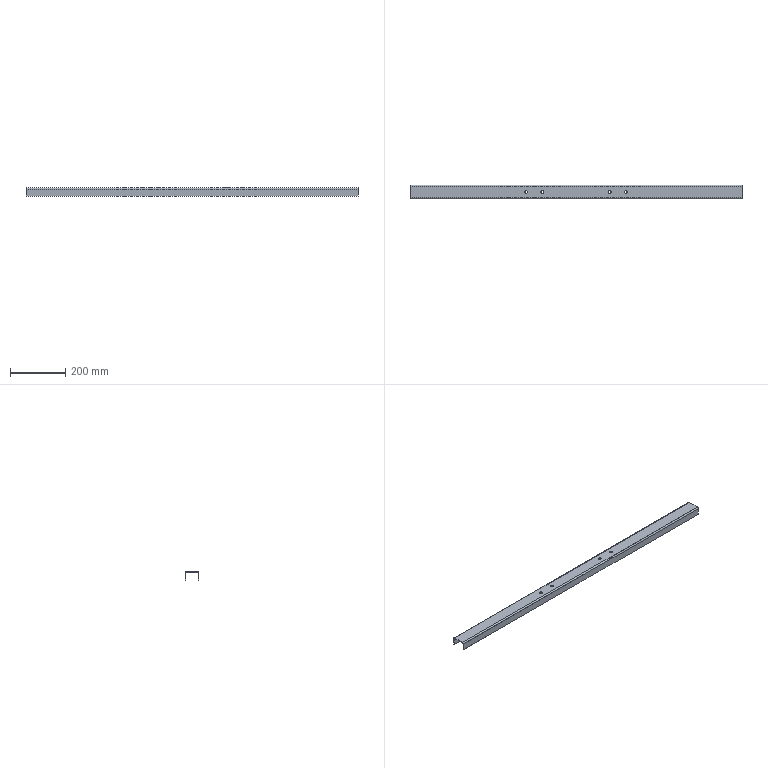Component | SolidWorks | 50x30x2ColdBentEqualAngleSteel1200mm-1 | 1 solid | 22 faces | box 1200 x 50 x 30 mm | volume 245531 mm3 | cylinder 12 | plane 10 | commonest cylinder face diameters 10 x10 6 x2
build123d program:
from build123d import *

# Parameters (mm, degrees)
BOSS_EXTRUDE1_DEPTH = 1200
SKETCH2_R           = 5
CUT_EXTRUDE1_DEPTH  = 10


with BuildPart() as part:
    # Sketch1 → Boss-Extrude1 (new body)
    with BuildSketch(Plane(origin=(0, 0, 0), x_dir=(0, 0, -1), z_dir=(1, 0, 0))):
        with BuildLine():
            Line((0, 5), (0, 45))
            ThreePointArc((0, 45), (1.464, 48.536), (5, 50))
            Line((5, 50), (30, 50))
            Line((30, 50), (30, 48))
            Line((30, 48), (5, 48))
            ThreePointArc((5, 48), (2.879, 47.121), (2, 45))
            Line((2, 45), (2, 5))
            ThreePointArc((2, 5), (2.879, 2.879), (5, 2))
            Line((5, 2), (30, 2))
            Line((30, 2), (30, 0))
            Line((30, 0), (5, 0))
            ThreePointArc((5, 0), (1.464, 1.464), (0, 5))
        make_face()
    extrude(amount=BOSS_EXTRUDE1_DEPTH)

    # Sketch2 → Cut-Extrude1 (cut)
    with BuildSketch(Plane.XY):
        with Locations((420, 25)):
            Circle(SKETCH2_R)
        with Locations((478, 25)):
            Circle(SKETCH2_R)
    cut_extrude1 = extrude(amount=-CUT_EXTRUDE1_DEPTH, mode=Mode.SUBTRACT)

    # Mirror2: Cut-Extrude1 across plane
    add(cut_extrude1.mirror(Plane.ZY.offset(-600)), mode=Mode.SUBTRACT)


solid = part.part

# Placed as in the assembly
solid = solid.moved(Location((-574.371, -297.9, 415), (0, 0, 0)))
STEP:
#1=COLOUR_RGB('',0.7922,0.8196,0.9333);
#2=FILL_AREA_STYLE_COLOUR('',#1);
#3=FILL_AREA_STYLE('',(#2));
#4=SURFACE_STYLE_FILL_AREA(#3);
#5=SURFACE_SIDE_STYLE('',(#4));
#6=SURFACE_STYLE_USAGE(.BOTH.,#5);
#7=PRESENTATION_STYLE_ASSIGNMENT((#6));
#8=CARTESIAN_POINT('',(8.292,-10.744,16.26));
#9=VERTEX_POINT('',#8);
#10=CARTESIAN_POINT('',(7.899,-10.744,16.26));
#11=VERTEX_POINT('',#10);
#12=CARTESIAN_POINT('',(8.096,-10.744,16.26));
#13=DIRECTION('',(0.,0.,-1.));
#14=DIRECTION('',(1.,0.,0.));
#15=AXIS2_PLACEMENT_3D('',#12,#13,#14);
#16=CIRCLE('',#15,0.1969);
#17=EDGE_CURVE('',#9,#11,#16,.T.);
#18=ORIENTED_EDGE('',*,*,#17,.T.);
#19=CARTESIAN_POINT('',(7.899,-10.744,16.339));
#20=VERTEX_POINT('',#19);
#21=CARTESIAN_POINT('',(7.899,-10.744,15.945));
#22=DIRECTION('',(0.,0.,1.));
#23=VECTOR('',#22,39.37);
#24=LINE('',#21,#23);
#25=EDGE_CURVE('',#11,#20,#24,.T.);
#26=ORIENTED_EDGE('',*,*,#25,.T.);
#27=CARTESIAN_POINT('',(8.292,-10.744,16.339));
#28=VERTEX_POINT('',#27);
#29=CARTESIAN_POINT('',(8.096,-10.744,16.339));
#30=DIRECTION('',(0.,0.,-1.));
#31=DIRECTION('',(-1.,0.,0.));
#32=AXIS2_PLACEMENT_3D('',#29,#30,#31);
#33=CIRCLE('',#32,0.1969);
#34=EDGE_CURVE('',#28,#20,#33,.T.);
#35=ORIENTED_EDGE('',*,*,#34,.F.);
#36=CARTESIAN_POINT('',(8.292,-10.744,15.945));
#37=DIRECTION('',(0.,0.,1.));
#38=VECTOR('',#37,39.37);
#39=LINE('',#36,#38);
#40=EDGE_CURVE('',#9,#28,#39,.T.);
#41=ORIENTED_EDGE('',*,*,#40,.F.);
#42=EDGE_LOOP('',(#18,#26,#35,#41));
#43=FACE_OUTER_BOUND('',#42,.T.);
#44=CARTESIAN_POINT('',(8.096,-10.744,15.945));
#45=DIRECTION('',(0.,0.,1.));
#46=DIRECTION('',(1.,0.,0.));
#47=AXIS2_PLACEMENT_3D('',#44,#45,#46);
#48=CYLINDRICAL_SURFACE('',#47,0.1969);
#49=ADVANCED_FACE('',(#43),#48,.F.);
#50=CARTESIAN_POINT('',(6.009,-10.744,16.26));
#51=VERTEX_POINT('',#50);
#52=CARTESIAN_POINT('',(5.615,-10.744,16.26));
#53=VERTEX_POINT('',#52);
#54=CARTESIAN_POINT('',(5.812,-10.744,16.26));
#55=DIRECTION('',(0.,0.,-1.));
#56=DIRECTION('',(1.,0.,0.));
#57=AXIS2_PLACEMENT_3D('',#54,#55,#56);
#58=CIRCLE('',#57,0.1969);
#59=EDGE_CURVE('',#51,#53,#58,.T.);
#60=ORIENTED_EDGE('',*,*,#59,.T.);
#61=CARTESIAN_POINT('',(5.615,-10.744,16.339));
#62=VERTEX_POINT('',#61);
#63=CARTESIAN_POINT('',(5.615,-10.744,15.945));
#64=DIRECTION('',(0.,0.,1.));
#65=VECTOR('',#64,39.37);
#66=LINE('',#63,#65);
#67=EDGE_CURVE('',#53,#62,#66,.T.);
#68=ORIENTED_EDGE('',*,*,#67,.T.);
#69=CARTESIAN_POINT('',(6.009,-10.744,16.339));
#70=VERTEX_POINT('',#69);
#71=CARTESIAN_POINT('',(5.812,-10.744,16.339));
#72=DIRECTION('',(0.,0.,-1.));
#73=DIRECTION('',(-1.,0.,0.));
#74=AXIS2_PLACEMENT_3D('',#71,#72,#73);
#75=CIRCLE('',#74,0.1969);
#76=EDGE_CURVE('',#70,#62,#75,.T.);
#77=ORIENTED_EDGE('',*,*,#76,.F.);
#78=CARTESIAN_POINT('',(6.009,-10.744,15.945));
#79=DIRECTION('',(0.,0.,1.));
#80=VECTOR('',#79,39.37);
#81=LINE('',#78,#80);
#82=EDGE_CURVE('',#51,#70,#81,.T.);
#83=ORIENTED_EDGE('',*,*,#82,.F.);
#84=EDGE_LOOP('',(#60,#68,#77,#83));
#85=FACE_OUTER_BOUND('',#84,.T.);
#86=CARTESIAN_POINT('',(5.812,-10.744,15.945));
#87=DIRECTION('',(0.,0.,1.));
#88=DIRECTION('',(1.,0.,0.));
#89=AXIS2_PLACEMENT_3D('',#86,#87,#88);
#90=CYLINDRICAL_SURFACE('',#89,0.1969);
#91=ADVANCED_FACE('',(#85),#90,.F.);
#92=CARTESIAN_POINT('',(-6.274,-10.744,16.26));
#93=VERTEX_POINT('',#92);
#94=CARTESIAN_POINT('',(-5.881,-10.744,16.26));
#95=VERTEX_POINT('',#94);
#96=CARTESIAN_POINT('',(-6.078,-10.744,16.26));
#97=DIRECTION('',(0.,0.,1.));
#98=DIRECTION('',(1.,0.,0.));
#99=AXIS2_PLACEMENT_3D('',#96,#97,#98);
#100=CIRCLE('',#99,0.1969);
#101=EDGE_CURVE('',#93,#95,#100,.T.);
#102=ORIENTED_EDGE('',*,*,#101,.F.);
#103=CARTESIAN_POINT('',(-6.274,-10.744,16.339));
#104=VERTEX_POINT('',#103);
#105=CARTESIAN_POINT('',(-6.274,-10.744,15.945));
#106=DIRECTION('',(0.,0.,1.));
#107=VECTOR('',#106,39.37);
#108=LINE('',#105,#107);
#109=EDGE_CURVE('',#93,#104,#108,.T.);
#110=ORIENTED_EDGE('',*,*,#109,.T.);
#111=CARTESIAN_POINT('',(-5.881,-10.744,16.339));
#112=VERTEX_POINT('',#111);
#113=CARTESIAN_POINT('',(-6.078,-10.744,16.339));
#114=DIRECTION('',(0.,0.,1.));
#115=DIRECTION('',(1.,0.,0.));
#116=AXIS2_PLACEMENT_3D('',#113,#114,#115);
#117=CIRCLE('',#116,0.1969);
#118=EDGE_CURVE('',#104,#112,#117,.T.);
#119=ORIENTED_EDGE('',*,*,#118,.T.);
#120=CARTESIAN_POINT('',(-5.881,-10.744,15.945));
#121=DIRECTION('',(0.,0.,1.));
#122=VECTOR('',#121,39.37);
#123=LINE('',#120,#122);
#124=EDGE_CURVE('',#95,#112,#123,.T.);
#125=ORIENTED_EDGE('',*,*,#124,.F.);
#126=EDGE_LOOP('',(#102,#110,#119,#125));
#127=FACE_OUTER_BOUND('',#126,.T.);
#128=CARTESIAN_POINT('',(-6.078,-10.744,15.945));
#129=DIRECTION('',(0.,0.,1.));
#130=DIRECTION('',(1.,0.,0.));
#131=AXIS2_PLACEMENT_3D('',#128,#129,#130);
#132=CYLINDRICAL_SURFACE('',#131,0.1969);
#133=ADVANCED_FACE('',(#127),#132,.F.);
#134=CARTESIAN_POINT('',(-3.991,-10.744,16.26));
#135=VERTEX_POINT('',#134);
#136=CARTESIAN_POINT('',(-3.597,-10.744,16.26));
#137=VERTEX_POINT('',#136);
#138=CARTESIAN_POINT('',(-3.794,-10.744,16.26));
#139=DIRECTION('',(0.,0.,1.));
#140=DIRECTION('',(1.,0.,0.));
#141=AXIS2_PLACEMENT_3D('',#138,#139,#140);
#142=CIRCLE('',#141,0.1969);
#143=EDGE_CURVE('',#135,#137,#142,.T.);
#144=ORIENTED_EDGE('',*,*,#143,.F.);
#145=CARTESIAN_POINT('',(-3.991,-10.744,16.339));
#146=VERTEX_POINT('',#145);
#147=CARTESIAN_POINT('',(-3.991,-10.744,15.945));
#148=DIRECTION('',(0.,0.,1.));
#149=VECTOR('',#148,39.37);
#150=LINE('',#147,#149);
#151=EDGE_CURVE('',#135,#146,#150,.T.);
#152=ORIENTED_EDGE('',*,*,#151,.T.);
#153=CARTESIAN_POINT('',(-3.597,-10.744,16.339));
#154=VERTEX_POINT('',#153);
#155=CARTESIAN_POINT('',(-3.794,-10.744,16.339));
#156=DIRECTION('',(0.,0.,1.));
#157=DIRECTION('',(1.,0.,0.));
#158=AXIS2_PLACEMENT_3D('',#155,#156,#157);
#159=CIRCLE('',#158,0.1969);
#160=EDGE_CURVE('',#146,#154,#159,.T.);
#161=ORIENTED_EDGE('',*,*,#160,.T.);
#162=CARTESIAN_POINT('',(-3.597,-10.744,15.945));
#163=DIRECTION('',(0.,0.,1.));
#164=VECTOR('',#163,39.37);
#165=LINE('',#162,#164);
#166=EDGE_CURVE('',#137,#154,#165,.T.);
#167=ORIENTED_EDGE('',*,*,#166,.F.);
#168=EDGE_LOOP('',(#144,#152,#161,#167));
#169=FACE_OUTER_BOUND('',#168,.T.);
#170=CARTESIAN_POINT('',(-3.794,-10.744,15.945));
#171=DIRECTION('',(0.,0.,1.));
#172=DIRECTION('',(1.,0.,0.));
#173=AXIS2_PLACEMENT_3D('',#170,#171,#172);
#174=CYLINDRICAL_SURFACE('',#173,0.1969);
#175=ADVANCED_FACE('',(#169),#174,.F.);
#176=CARTESIAN_POINT('',(-22.613,-9.76,16.142));
#177=VERTEX_POINT('',#176);
#178=CARTESIAN_POINT('',(-22.613,-9.957,16.339));
#179=VERTEX_POINT('',#178);
#180=CARTESIAN_POINT('',(-22.613,-9.957,16.142));
#181=DIRECTION('',(1.,0.,0.));
#182=DIRECTION('',(0.,0.,1.));
#183=AXIS2_PLACEMENT_3D('',#180,#181,#182);
#184=CIRCLE('',#183,0.1969);
#185=EDGE_CURVE('',#177,#179,#184,.T.);
#186=ORIENTED_EDGE('',*,*,#185,.T.);
#187=CARTESIAN_POINT('',(24.631,-9.957,16.339));
#188=VERTEX_POINT('',#187);
#189=CARTESIAN_POINT('',(24.631,-9.957,16.339));
#190=DIRECTION('',(-1.,0.,0.));
#191=VECTOR('',#190,39.37);
#192=LINE('',#189,#191);
#193=EDGE_CURVE('',#188,#179,#192,.T.);
#194=ORIENTED_EDGE('',*,*,#193,.F.);
#195=CARTESIAN_POINT('',(24.631,-9.76,16.142));
#196=VERTEX_POINT('',#195);
#197=CARTESIAN_POINT('',(24.631,-9.957,16.142));
#198=DIRECTION('',(1.,0.,0.));
#199=DIRECTION('',(0.,0.,1.));
#200=AXIS2_PLACEMENT_3D('',#197,#198,#199);
#201=CIRCLE('',#200,0.1969);
#202=EDGE_CURVE('',#196,#188,#201,.T.);
#203=ORIENTED_EDGE('',*,*,#202,.F.);
#204=CARTESIAN_POINT('',(24.631,-9.76,16.142));
#205=DIRECTION('',(-1.,0.,0.));
#206=VECTOR('',#205,39.37);
#207=LINE('',#204,#206);
#208=EDGE_CURVE('',#196,#177,#207,.T.);
#209=ORIENTED_EDGE('',*,*,#208,.T.);
#210=EDGE_LOOP('',(#186,#194,#203,#209));
#211=FACE_OUTER_BOUND('',#210,.T.);
#212=CARTESIAN_POINT('',(24.631,-9.957,16.142));
#213=DIRECTION('',(-1.,0.,0.));
#214=DIRECTION('',(0.,0.,1.));
#215=AXIS2_PLACEMENT_3D('',#212,#213,#214);
#216=CYLINDRICAL_SURFACE('',#215,0.1969);
#217=ADVANCED_FACE('',(#211),#216,.T.);
#218=ORIENTED_EDGE('',*,*,#34,.T.);
#219=CARTESIAN_POINT('',(8.096,-10.744,16.339));
#220=DIRECTION('',(0.,0.,-1.));
#221=DIRECTION('',(-1.,0.,0.));
#222=AXIS2_PLACEMENT_3D('',#219,#220,#221);
#223=CIRCLE('',#222,0.1969);
#224=EDGE_CURVE('',#20,#28,#223,.T.);
#225=ORIENTED_EDGE('',*,*,#224,.T.);
#226=EDGE_LOOP('',(#218,#225));
#227=FACE_BOUND('',#226,.T.);
#228=ORIENTED_EDGE('',*,*,#76,.T.);
#229=CARTESIAN_POINT('',(5.812,-10.744,16.339));
#230=DIRECTION('',(0.,0.,-1.));
#231=DIRECTION('',(-1.,0.,0.));
#232=AXIS2_PLACEMENT_3D('',#229,#230,#231);
#233=CIRCLE('',#232,0.1969);
#234=EDGE_CURVE('',#62,#70,#233,.T.);
#235=ORIENTED_EDGE('',*,*,#234,.T.);
#236=EDGE_LOOP('',(#228,#235));
#237=FACE_BOUND('',#236,.T.);
#238=CARTESIAN_POINT('',(-6.078,-10.744,16.339));
#239=DIRECTION('',(0.,0.,1.));
#240=DIRECTION('',(1.,0.,0.));
#241=AXIS2_PLACEMENT_3D('',#238,#239,#240);
#242=CIRCLE('',#241,0.1969);
#243=EDGE_CURVE('',#112,#104,#242,.T.);
#244=ORIENTED_EDGE('',*,*,#243,.F.);
#245=ORIENTED_EDGE('',*,*,#118,.F.);
#246=EDGE_LOOP('',(#244,#245));
#247=FACE_BOUND('',#246,.T.);
#248=CARTESIAN_POINT('',(-3.794,-10.744,16.339));
#249=DIRECTION('',(0.,0.,1.));
#250=DIRECTION('',(1.,0.,0.));
#251=AXIS2_PLACEMENT_3D('',#248,#249,#250);
#252=CIRCLE('',#251,0.1969);
#253=EDGE_CURVE('',#154,#146,#252,.T.);
#254=ORIENTED_EDGE('',*,*,#253,.F.);
#255=ORIENTED_EDGE('',*,*,#160,.F.);
#256=EDGE_LOOP('',(#254,#255));
#257=FACE_BOUND('',#256,.T.);
#258=CARTESIAN_POINT('',(-22.613,-11.532,16.339));
#259=VERTEX_POINT('',#258);
#260=CARTESIAN_POINT('',(-22.613,-11.532,16.339));
#261=DIRECTION('',(0.,-1.,0.));
#262=VECTOR('',#261,39.37);
#263=LINE('',#260,#262);
#264=EDGE_CURVE('',#179,#259,#263,.T.);
#265=ORIENTED_EDGE('',*,*,#264,.T.);
#266=CARTESIAN_POINT('',(24.631,-11.532,16.339));
#267=VERTEX_POINT('',#266);
#268=CARTESIAN_POINT('',(24.631,-11.532,16.339));
#269=DIRECTION('',(-1.,0.,0.));
#270=VECTOR('',#269,39.37);
#271=LINE('',#268,#270);
#272=EDGE_CURVE('',#267,#259,#271,.T.);
#273=ORIENTED_EDGE('',*,*,#272,.F.);
#274=CARTESIAN_POINT('',(24.631,-11.532,16.339));
#275=DIRECTION('',(0.,-1.,0.));
#276=VECTOR('',#275,39.37);
#277=LINE('',#274,#276);
#278=EDGE_CURVE('',#188,#267,#277,.T.);
#279=ORIENTED_EDGE('',*,*,#278,.F.);
#280=ORIENTED_EDGE('',*,*,#193,.T.);
#281=EDGE_LOOP('',(#265,#273,#279,#280));
#282=FACE_OUTER_BOUND('',#281,.T.);
#283=CARTESIAN_POINT('',(24.631,-11.532,16.339));
#284=DIRECTION('',(0.,0.,-1.));
#285=DIRECTION('',(-1.,0.,0.));
#286=AXIS2_PLACEMENT_3D('',#283,#284,#285);
#287=PLANE('',#286);
#288=ADVANCED_FACE('',(#227,#237,#247,#257,#282),#287,.F.);
#289=CARTESIAN_POINT('',(-22.613,-11.728,16.142));
#290=VERTEX_POINT('',#289);
#291=CARTESIAN_POINT('',(-22.613,-11.532,16.142));
#292=DIRECTION('',(1.,0.,0.));
#293=DIRECTION('',(0.,0.,-1.));
#294=AXIS2_PLACEMENT_3D('',#291,#292,#293);
#295=CIRCLE('',#294,0.1969);
#296=EDGE_CURVE('',#259,#290,#295,.T.);
#297=ORIENTED_EDGE('',*,*,#296,.T.);
#298=CARTESIAN_POINT('',(24.631,-11.728,16.142));
#299=VERTEX_POINT('',#298);
#300=CARTESIAN_POINT('',(24.631,-11.728,16.142));
#301=DIRECTION('',(-1.,0.,0.));
#302=VECTOR('',#301,39.37);
#303=LINE('',#300,#302);
#304=EDGE_CURVE('',#299,#290,#303,.T.);
#305=ORIENTED_EDGE('',*,*,#304,.F.);
#306=CARTESIAN_POINT('',(24.631,-11.532,16.142));
#307=DIRECTION('',(1.,0.,0.));
#308=DIRECTION('',(0.,0.,-1.));
#309=AXIS2_PLACEMENT_3D('',#306,#307,#308);
#310=CIRCLE('',#309,0.1969);
#311=EDGE_CURVE('',#267,#299,#310,.T.);
#312=ORIENTED_EDGE('',*,*,#311,.F.);
#313=ORIENTED_EDGE('',*,*,#272,.T.);
#314=EDGE_LOOP('',(#297,#305,#312,#313));
#315=FACE_OUTER_BOUND('',#314,.T.);
#316=CARTESIAN_POINT('',(24.631,-11.532,16.142));
#317=DIRECTION('',(-1.,0.,0.));
#318=DIRECTION('',(0.,0.,1.));
#319=AXIS2_PLACEMENT_3D('',#316,#317,#318);
#320=CYLINDRICAL_SURFACE('',#319,0.1969);
#321=ADVANCED_FACE('',(#315),#320,.T.);
#322=CARTESIAN_POINT('',(-22.613,-11.728,15.157));
#323=VERTEX_POINT('',#322);
#324=CARTESIAN_POINT('',(-22.613,-11.728,16.142));
#325=DIRECTION('',(0.,0.,-1.));
#326=VECTOR('',#325,39.37);
#327=LINE('',#324,#326);
#328=EDGE_CURVE('',#290,#323,#327,.T.);
#329=ORIENTED_EDGE('',*,*,#328,.T.);
#330=CARTESIAN_POINT('',(24.631,-11.728,15.157));
#331=VERTEX_POINT('',#330);
#332=CARTESIAN_POINT('',(24.631,-11.728,15.157));
#333=DIRECTION('',(-1.,0.,0.));
#334=VECTOR('',#333,39.37);
#335=LINE('',#332,#334);
#336=EDGE_CURVE('',#331,#323,#335,.T.);
#337=ORIENTED_EDGE('',*,*,#336,.F.);
#338=CARTESIAN_POINT('',(24.631,-11.728,16.142));
#339=DIRECTION('',(0.,0.,-1.));
#340=VECTOR('',#339,39.37);
#341=LINE('',#338,#340);
#342=EDGE_CURVE('',#299,#331,#341,.T.);
#343=ORIENTED_EDGE('',*,*,#342,.F.);
#344=ORIENTED_EDGE('',*,*,#304,.T.);
#345=EDGE_LOOP('',(#329,#337,#343,#344));
#346=FACE_OUTER_BOUND('',#345,.T.);
#347=CARTESIAN_POINT('',(24.631,-11.728,16.142));
#348=DIRECTION('',(0.,1.,0.));
#349=DIRECTION('',(0.,0.,1.));
#350=AXIS2_PLACEMENT_3D('',#347,#348,#349);
#351=PLANE('',#350);
#352=ADVANCED_FACE('',(#346),#351,.F.);
#353=CARTESIAN_POINT('',(-22.613,-11.65,15.157));
#354=VERTEX_POINT('',#353);
#355=CARTESIAN_POINT('',(-22.613,-11.65,15.157));
#356=DIRECTION('',(0.,1.,0.));
#357=VECTOR('',#356,39.37);
#358=LINE('',#355,#357);
#359=EDGE_CURVE('',#323,#354,#358,.T.);
#360=ORIENTED_EDGE('',*,*,#359,.T.);
#361=CARTESIAN_POINT('',(24.631,-11.65,15.157));
#362=VERTEX_POINT('',#361);
#363=CARTESIAN_POINT('',(24.631,-11.65,15.157));
#364=DIRECTION('',(-1.,0.,0.));
#365=VECTOR('',#364,39.37);
#366=LINE('',#363,#365);
#367=EDGE_CURVE('',#362,#354,#366,.T.);
#368=ORIENTED_EDGE('',*,*,#367,.F.);
#369=CARTESIAN_POINT('',(24.631,-11.65,15.157));
#370=DIRECTION('',(0.,1.,0.));
#371=VECTOR('',#370,39.37);
#372=LINE('',#369,#371);
#373=EDGE_CURVE('',#331,#362,#372,.T.);
#374=ORIENTED_EDGE('',*,*,#373,.F.);
#375=ORIENTED_EDGE('',*,*,#336,.T.);
#376=EDGE_LOOP('',(#360,#368,#374,#375));
#377=FACE_OUTER_BOUND('',#376,.T.);
#378=CARTESIAN_POINT('',(24.631,-11.65,15.157));
#379=DIRECTION('',(0.,0.,1.));
#380=DIRECTION('',(1.,0.,0.));
#381=AXIS2_PLACEMENT_3D('',#378,#379,#380);
#382=PLANE('',#381);
#383=ADVANCED_FACE('',(#377),#382,.F.);
#384=CARTESIAN_POINT('',(-22.613,-11.65,16.142));
#385=VERTEX_POINT('',#384);
#386=CARTESIAN_POINT('',(-22.613,-11.65,16.142));
#387=DIRECTION('',(0.,0.,1.));
#388=VECTOR('',#387,39.37);
#389=LINE('',#386,#388);
#390=EDGE_CURVE('',#354,#385,#389,.T.);
#391=ORIENTED_EDGE('',*,*,#390,.T.);
#392=CARTESIAN_POINT('',(24.631,-11.65,16.142));
#393=VERTEX_POINT('',#392);
#394=CARTESIAN_POINT('',(24.631,-11.65,16.142));
#395=DIRECTION('',(-1.,0.,0.));
#396=VECTOR('',#395,39.37);
#397=LINE('',#394,#396);
#398=EDGE_CURVE('',#393,#385,#397,.T.);
#399=ORIENTED_EDGE('',*,*,#398,.F.);
#400=CARTESIAN_POINT('',(24.631,-11.65,16.142));
#401=DIRECTION('',(0.,0.,1.));
#402=VECTOR('',#401,39.37);
#403=LINE('',#400,#402);
#404=EDGE_CURVE('',#362,#393,#403,.T.);
#405=ORIENTED_EDGE('',*,*,#404,.F.);
#406=ORIENTED_EDGE('',*,*,#367,.T.);
#407=EDGE_LOOP('',(#391,#399,#405,#406));
#408=FACE_OUTER_BOUND('',#407,.T.);
#409=CARTESIAN_POINT('',(24.631,-11.65,16.142));
#410=DIRECTION('',(0.,-1.,0.));
#411=DIRECTION('',(0.,0.,-1.));
#412=AXIS2_PLACEMENT_3D('',#409,#410,#411);
#413=PLANE('',#412);
#414=ADVANCED_FACE('',(#408),#413,.F.);
#415=CARTESIAN_POINT('',(-22.613,-11.532,16.26));
#416=VERTEX_POINT('',#415);
#417=CARTESIAN_POINT('',(-22.613,-11.532,16.142));
#418=DIRECTION('',(-1.,0.,0.));
#419=DIRECTION('',(0.,0.,-1.));
#420=AXIS2_PLACEMENT_3D('',#417,#418,#419);
#421=CIRCLE('',#420,0.1181);
#422=EDGE_CURVE('',#385,#416,#421,.T.);
#423=ORIENTED_EDGE('',*,*,#422,.T.);
#424=CARTESIAN_POINT('',(24.631,-11.532,16.26));
#425=VERTEX_POINT('',#424);
#426=CARTESIAN_POINT('',(24.631,-11.532,16.26));
#427=DIRECTION('',(-1.,0.,0.));
#428=VECTOR('',#427,39.37);
#429=LINE('',#426,#428);
#430=EDGE_CURVE('',#425,#416,#429,.T.);
#431=ORIENTED_EDGE('',*,*,#430,.F.);
#432=CARTESIAN_POINT('',(24.631,-11.532,16.142));
#433=DIRECTION('',(-1.,0.,0.));
#434=DIRECTION('',(0.,0.,-1.));
#435=AXIS2_PLACEMENT_3D('',#432,#433,#434);
#436=CIRCLE('',#435,0.1181);
#437=EDGE_CURVE('',#393,#425,#436,.T.);
#438=ORIENTED_EDGE('',*,*,#437,.F.);
#439=ORIENTED_EDGE('',*,*,#398,.T.);
#440=EDGE_LOOP('',(#423,#431,#438,#439));
#441=FACE_OUTER_BOUND('',#440,.T.);
#442=CARTESIAN_POINT('',(24.631,-11.532,16.142));
#443=DIRECTION('',(-1.,0.,0.));
#444=DIRECTION('',(0.,0.,1.));
#445=AXIS2_PLACEMENT_3D('',#442,#443,#444);
#446=CYLINDRICAL_SURFACE('',#445,0.1181);
#447=ADVANCED_FACE('',(#441),#446,.F.);
#448=ORIENTED_EDGE('',*,*,#17,.F.);
#449=CARTESIAN_POINT('',(8.096,-10.744,16.26));
#450=DIRECTION('',(0.,0.,-1.));
#451=DIRECTION('',(1.,0.,0.));
#452=AXIS2_PLACEMENT_3D('',#449,#450,#451);
#453=CIRCLE('',#452,0.1969);
#454=EDGE_CURVE('',#11,#9,#453,.T.);
#455=ORIENTED_EDGE('',*,*,#454,.F.);
#456=EDGE_LOOP('',(#448,#455));
#457=FACE_BOUND('',#456,.T.);
#458=ORIENTED_EDGE('',*,*,#59,.F.);
#459=CARTESIAN_POINT('',(5.812,-10.744,16.26));
#460=DIRECTION('',(0.,0.,-1.));
#461=DIRECTION('',(1.,0.,0.));
#462=AXIS2_PLACEMENT_3D('',#459,#460,#461);
#463=CIRCLE('',#462,0.1969);
#464=EDGE_CURVE('',#53,#51,#463,.T.);
#465=ORIENTED_EDGE('',*,*,#464,.F.);
#466=EDGE_LOOP('',(#458,#465));
#467=FACE_BOUND('',#466,.T.);
#468=CARTESIAN_POINT('',(-6.078,-10.744,16.26));
#469=DIRECTION('',(0.,0.,1.));
#470=DIRECTION('',(1.,0.,0.));
#471=AXIS2_PLACEMENT_3D('',#468,#469,#470);
#472=CIRCLE('',#471,0.1969);
#473=EDGE_CURVE('',#95,#93,#472,.T.);
#474=ORIENTED_EDGE('',*,*,#473,.T.);
#475=ORIENTED_EDGE('',*,*,#101,.T.);
#476=EDGE_LOOP('',(#474,#475));
#477=FACE_BOUND('',#476,.T.);
#478=CARTESIAN_POINT('',(-3.794,-10.744,16.26));
#479=DIRECTION('',(0.,0.,1.));
#480=DIRECTION('',(1.,0.,0.));
#481=AXIS2_PLACEMENT_3D('',#478,#479,#480);
#482=CIRCLE('',#481,0.1969);
#483=EDGE_CURVE('',#137,#135,#482,.T.);
#484=ORIENTED_EDGE('',*,*,#483,.T.);
#485=ORIENTED_EDGE('',*,*,#143,.T.);
#486=EDGE_LOOP('',(#484,#485));
#487=FACE_BOUND('',#486,.T.);
#488=CARTESIAN_POINT('',(-22.613,-9.957,16.26));
#489=VERTEX_POINT('',#488);
#490=CARTESIAN_POINT('',(-22.613,-11.532,16.26));
#491=DIRECTION('',(0.,1.,0.));
#492=VECTOR('',#491,39.37);
#493=LINE('',#490,#492);
#494=EDGE_CURVE('',#416,#489,#493,.T.);
#495=ORIENTED_EDGE('',*,*,#494,.T.);
#496=CARTESIAN_POINT('',(24.631,-9.957,16.26));
#497=VERTEX_POINT('',#496);
#498=CARTESIAN_POINT('',(24.631,-9.957,16.26));
#499=DIRECTION('',(-1.,0.,0.));
#500=VECTOR('',#499,39.37);
#501=LINE('',#498,#500);
#502=EDGE_CURVE('',#497,#489,#501,.T.);
#503=ORIENTED_EDGE('',*,*,#502,.F.);
#504=CARTESIAN_POINT('',(24.631,-11.532,16.26));
#505=DIRECTION('',(0.,1.,0.));
#506=VECTOR('',#505,39.37);
#507=LINE('',#504,#506);
#508=EDGE_CURVE('',#425,#497,#507,.T.);
#509=ORIENTED_EDGE('',*,*,#508,.F.);
#510=ORIENTED_EDGE('',*,*,#430,.T.);
#511=EDGE_LOOP('',(#495,#503,#509,#510));
#512=FACE_OUTER_BOUND('',#511,.T.);
#513=CARTESIAN_POINT('',(24.631,-11.532,16.26));
#514=DIRECTION('',(0.,0.,1.));
#515=DIRECTION('',(1.,0.,0.));
#516=AXIS2_PLACEMENT_3D('',#513,#514,#515);
#517=PLANE('',#516);
#518=ADVANCED_FACE('',(#457,#467,#477,#487,#512),#517,.F.);
#519=CARTESIAN_POINT('',(-22.613,-9.839,16.142));
#520=VERTEX_POINT('',#519);
#521=CARTESIAN_POINT('',(-22.613,-9.957,16.142));
#522=DIRECTION('',(-1.,0.,0.));
#523=DIRECTION('',(0.,0.,1.));
#524=AXIS2_PLACEMENT_3D('',#521,#522,#523);
#525=CIRCLE('',#524,0.1181);
#526=EDGE_CURVE('',#489,#520,#525,.T.);
#527=ORIENTED_EDGE('',*,*,#526,.T.);
#528=CARTESIAN_POINT('',(24.631,-9.839,16.142));
#529=VERTEX_POINT('',#528);
#530=CARTESIAN_POINT('',(24.631,-9.839,16.142));
#531=DIRECTION('',(-1.,0.,0.));
#532=VECTOR('',#531,39.37);
#533=LINE('',#530,#532);
#534=EDGE_CURVE('',#529,#520,#533,.T.);
#535=ORIENTED_EDGE('',*,*,#534,.F.);
#536=CARTESIAN_POINT('',(24.631,-9.957,16.142));
#537=DIRECTION('',(-1.,0.,0.));
#538=DIRECTION('',(0.,0.,1.));
#539=AXIS2_PLACEMENT_3D('',#536,#537,#538);
#540=CIRCLE('',#539,0.1181);
#541=EDGE_CURVE('',#497,#529,#540,.T.);
#542=ORIENTED_EDGE('',*,*,#541,.F.);
#543=ORIENTED_EDGE('',*,*,#502,.T.);
#544=EDGE_LOOP('',(#527,#535,#542,#543));
#545=FACE_OUTER_BOUND('',#544,.T.);
#546=CARTESIAN_POINT('',(24.631,-9.957,16.142));
#547=DIRECTION('',(-1.,0.,0.));
#548=DIRECTION('',(0.,0.,1.));
#549=AXIS2_PLACEMENT_3D('',#546,#547,#548);
#550=CYLINDRICAL_SURFACE('',#549,0.1181);
#551=ADVANCED_FACE('',(#545),#550,.F.);
#552=CARTESIAN_POINT('',(-22.613,-9.839,15.157));
#553=VERTEX_POINT('',#552);
#554=CARTESIAN_POINT('',(-22.613,-9.839,16.142));
#555=DIRECTION('',(0.,0.,-1.));
#556=VECTOR('',#555,39.37);
#557=LINE('',#554,#556);
#558=EDGE_CURVE('',#520,#553,#557,.T.);
#559=ORIENTED_EDGE('',*,*,#558,.T.);
#560=CARTESIAN_POINT('',(24.631,-9.839,15.157));
#561=VERTEX_POINT('',#560);
#562=CARTESIAN_POINT('',(24.631,-9.839,15.157));
#563=DIRECTION('',(-1.,0.,0.));
#564=VECTOR('',#563,39.37);
#565=LINE('',#562,#564);
#566=EDGE_CURVE('',#561,#553,#565,.T.);
#567=ORIENTED_EDGE('',*,*,#566,.F.);
#568=CARTESIAN_POINT('',(24.631,-9.839,16.142));
#569=DIRECTION('',(0.,0.,-1.));
#570=VECTOR('',#569,39.37);
#571=LINE('',#568,#570);
#572=EDGE_CURVE('',#529,#561,#571,.T.);
#573=ORIENTED_EDGE('',*,*,#572,.F.);
#574=ORIENTED_EDGE('',*,*,#534,.T.);
#575=EDGE_LOOP('',(#559,#567,#573,#574));
#576=FACE_OUTER_BOUND('',#575,.T.);
#577=CARTESIAN_POINT('',(24.631,-9.839,16.142));
#578=DIRECTION('',(0.,1.,0.));
#579=DIRECTION('',(0.,0.,1.));
#580=AXIS2_PLACEMENT_3D('',#577,#578,#579);
#581=PLANE('',#580);
#582=ADVANCED_FACE('',(#576),#581,.F.);
#583=CARTESIAN_POINT('',(-22.613,-9.76,15.157));
#584=VERTEX_POINT('',#583);
#585=CARTESIAN_POINT('',(-22.613,-9.76,15.157));
#586=DIRECTION('',(0.,1.,0.));
#587=VECTOR('',#586,39.37);
#588=LINE('',#585,#587);
#589=EDGE_CURVE('',#553,#584,#588,.T.);
#590=ORIENTED_EDGE('',*,*,#589,.T.);
#591=CARTESIAN_POINT('',(24.631,-9.76,15.157));
#592=VERTEX_POINT('',#591);
#593=CARTESIAN_POINT('',(24.631,-9.76,15.157));
#594=DIRECTION('',(-1.,0.,0.));
#595=VECTOR('',#594,39.37);
#596=LINE('',#593,#595);
#597=EDGE_CURVE('',#592,#584,#596,.T.);
#598=ORIENTED_EDGE('',*,*,#597,.F.);
#599=CARTESIAN_POINT('',(24.631,-9.76,15.157));
#600=DIRECTION('',(0.,1.,0.));
#601=VECTOR('',#600,39.37);
#602=LINE('',#599,#601);
#603=EDGE_CURVE('',#561,#592,#602,.T.);
#604=ORIENTED_EDGE('',*,*,#603,.F.);
#605=ORIENTED_EDGE('',*,*,#566,.T.);
#606=EDGE_LOOP('',(#590,#598,#604,#605));
#607=FACE_OUTER_BOUND('',#606,.T.);
#608=CARTESIAN_POINT('',(24.631,-9.76,15.157));
#609=DIRECTION('',(0.,0.,1.));
#610=DIRECTION('',(1.,0.,0.));
#611=AXIS2_PLACEMENT_3D('',#608,#609,#610);
#612=PLANE('',#611);
#613=ADVANCED_FACE('',(#607),#612,.F.);
#614=CARTESIAN_POINT('',(-22.613,-9.76,16.142));
#615=DIRECTION('',(0.,0.,1.));
#616=VECTOR('',#615,39.37);
#617=LINE('',#614,#616);
#618=EDGE_CURVE('',#584,#177,#617,.T.);
#619=ORIENTED_EDGE('',*,*,#618,.T.);
#620=ORIENTED_EDGE('',*,*,#208,.F.);
#621=CARTESIAN_POINT('',(24.631,-9.76,16.142));
#622=DIRECTION('',(0.,0.,1.));
#623=VECTOR('',#622,39.37);
#624=LINE('',#621,#623);
#625=EDGE_CURVE('',#592,#196,#624,.T.);
#626=ORIENTED_EDGE('',*,*,#625,.F.);
#627=ORIENTED_EDGE('',*,*,#597,.T.);
#628=EDGE_LOOP('',(#619,#620,#626,#627));
#629=FACE_OUTER_BOUND('',#628,.T.);
#630=CARTESIAN_POINT('',(24.631,-9.76,16.142));
#631=DIRECTION('',(0.,-1.,0.));
#632=DIRECTION('',(0.,0.,-1.));
#633=AXIS2_PLACEMENT_3D('',#630,#631,#632);
#634=PLANE('',#633);
#635=ADVANCED_FACE('',(#629),#634,.F.);
#636=ORIENTED_EDGE('',*,*,#202,.T.);
#637=ORIENTED_EDGE('',*,*,#278,.T.);
#638=ORIENTED_EDGE('',*,*,#311,.T.);
#639=ORIENTED_EDGE('',*,*,#342,.T.);
#640=ORIENTED_EDGE('',*,*,#373,.T.);
#641=ORIENTED_EDGE('',*,*,#404,.T.);
#642=ORIENTED_EDGE('',*,*,#437,.T.);
#643=ORIENTED_EDGE('',*,*,#508,.T.);
#644=ORIENTED_EDGE('',*,*,#541,.T.);
#645=ORIENTED_EDGE('',*,*,#572,.T.);
#646=ORIENTED_EDGE('',*,*,#603,.T.);
#647=ORIENTED_EDGE('',*,*,#625,.T.);
#648=EDGE_LOOP('',(#636,#637,#638,#639,#640,#641,#642,#643,#644,#645,#646,#647));
#649=FACE_OUTER_BOUND('',#648,.T.);
#650=CARTESIAN_POINT('',(24.631,-9.957,16.142));
#651=DIRECTION('',(-1.,0.,0.));
#652=DIRECTION('',(0.,0.,1.));
#653=AXIS2_PLACEMENT_3D('',#650,#651,#652);
#654=PLANE('',#653);
#655=ADVANCED_FACE('',(#649),#654,.F.);
#656=ORIENTED_EDGE('',*,*,#185,.F.);
#657=ORIENTED_EDGE('',*,*,#618,.F.);
#658=ORIENTED_EDGE('',*,*,#589,.F.);
#659=ORIENTED_EDGE('',*,*,#558,.F.);
#660=ORIENTED_EDGE('',*,*,#526,.F.);
#661=ORIENTED_EDGE('',*,*,#494,.F.);
#662=ORIENTED_EDGE('',*,*,#422,.F.);
#663=ORIENTED_EDGE('',*,*,#390,.F.);
#664=ORIENTED_EDGE('',*,*,#359,.F.);
#665=ORIENTED_EDGE('',*,*,#328,.F.);
#666=ORIENTED_EDGE('',*,*,#296,.F.);
#667=ORIENTED_EDGE('',*,*,#264,.F.);
#668=EDGE_LOOP('',(#656,#657,#658,#659,#660,#661,#662,#663,#664,#665,#666,#667));
#669=FACE_OUTER_BOUND('',#668,.T.);
#670=CARTESIAN_POINT('',(-22.613,-9.957,16.142));
#671=DIRECTION('',(-1.,0.,0.));
#672=DIRECTION('',(0.,0.,1.));
#673=AXIS2_PLACEMENT_3D('',#670,#671,#672);
#674=PLANE('',#673);
#675=ADVANCED_FACE('',(#669),#674,.T.);
#676=ORIENTED_EDGE('',*,*,#151,.F.);
#677=ORIENTED_EDGE('',*,*,#483,.F.);
#678=ORIENTED_EDGE('',*,*,#166,.T.);
#679=ORIENTED_EDGE('',*,*,#253,.T.);
#680=EDGE_LOOP('',(#676,#677,#678,#679));
#681=FACE_OUTER_BOUND('',#680,.T.);
#682=CARTESIAN_POINT('',(-3.794,-10.744,15.945));
#683=DIRECTION('',(0.,0.,1.));
#684=DIRECTION('',(1.,0.,0.));
#685=AXIS2_PLACEMENT_3D('',#682,#683,#684);
#686=CYLINDRICAL_SURFACE('',#685,0.1969);
#687=ADVANCED_FACE('',(#681),#686,.F.);
#688=ORIENTED_EDGE('',*,*,#109,.F.);
#689=ORIENTED_EDGE('',*,*,#473,.F.);
#690=ORIENTED_EDGE('',*,*,#124,.T.);
#691=ORIENTED_EDGE('',*,*,#243,.T.);
#692=EDGE_LOOP('',(#688,#689,#690,#691));
#693=FACE_OUTER_BOUND('',#692,.T.);
#694=CARTESIAN_POINT('',(-6.078,-10.744,15.945));
#695=DIRECTION('',(0.,0.,1.));
#696=DIRECTION('',(1.,0.,0.));
#697=AXIS2_PLACEMENT_3D('',#694,#695,#696);
#698=CYLINDRICAL_SURFACE('',#697,0.1969);
#699=ADVANCED_FACE('',(#693),#698,.F.);
#700=ORIENTED_EDGE('',*,*,#67,.F.);
#701=ORIENTED_EDGE('',*,*,#464,.T.);
#702=ORIENTED_EDGE('',*,*,#82,.T.);
#703=ORIENTED_EDGE('',*,*,#234,.F.);
#704=EDGE_LOOP('',(#700,#701,#702,#703));
#705=FACE_OUTER_BOUND('',#704,.T.);
#706=CARTESIAN_POINT('',(5.812,-10.744,15.945));
#707=DIRECTION('',(0.,0.,1.));
#708=DIRECTION('',(1.,0.,0.));
#709=AXIS2_PLACEMENT_3D('',#706,#707,#708);
#710=CYLINDRICAL_SURFACE('',#709,0.1969);
#711=ADVANCED_FACE('',(#705),#710,.F.);
#712=ORIENTED_EDGE('',*,*,#25,.F.);
#713=ORIENTED_EDGE('',*,*,#454,.T.);
#714=ORIENTED_EDGE('',*,*,#40,.T.);
#715=ORIENTED_EDGE('',*,*,#224,.F.);
#716=EDGE_LOOP('',(#712,#713,#714,#715));
#717=FACE_OUTER_BOUND('',#716,.T.);
#718=CARTESIAN_POINT('',(8.096,-10.744,15.945));
#719=DIRECTION('',(0.,0.,1.));
#720=DIRECTION('',(1.,0.,0.));
#721=AXIS2_PLACEMENT_3D('',#718,#719,#720);
#722=CYLINDRICAL_SURFACE('',#721,0.1969);
#723=ADVANCED_FACE('',(#717),#722,.F.);
#724=CLOSED_SHELL('',(#49,#91,#133,#175,#217,#288,#321,#352,#383,#414,#447,#518,#551,#582,#613,#635,#655,#675,#687,#699,#711,#723));
#725=MANIFOLD_SOLID_BREP('',#724);
#726=STYLED_ITEM('',(#7),#725);
#727=PRESENTATION_LAYER_ASSIGNMENT('','',(#726));
#728=CARTESIAN_POINT('',(0.,0.,0.));
#729=DIRECTION('',(0.,0.,1.));
#730=DIRECTION('',(1.,0.,0.));
#731=AXIS2_PLACEMENT_3D('',#728,#729,#730);
#732=(LENGTH_UNIT()NAMED_UNIT(*)SI_UNIT($,.METRE.));
#733=LENGTH_MEASURE_WITH_UNIT(LENGTH_MEASURE(0.0254),#732);
#734=DIMENSIONAL_EXPONENTS(1.,0.,0.,0.,0.,0.,0.);
#735=(CONVERSION_BASED_UNIT('',#733)LENGTH_UNIT()NAMED_UNIT(#734));
#736=UNCERTAINTY_MEASURE_WITH_UNIT(LENGTH_MEASURE(0.00001),#735,'','');
#737=(NAMED_UNIT(*)PLANE_ANGLE_UNIT()SI_UNIT($,.RADIAN.));
#738=(NAMED_UNIT(*)SI_UNIT($,.STERADIAN.)SOLID_ANGLE_UNIT());
#739=(GEOMETRIC_REPRESENTATION_CONTEXT(3)GLOBAL_UNCERTAINTY_ASSIGNED_CONTEXT((#736))GLOBAL_UNIT_ASSIGNED_CONTEXT((#735,#737,#738))REPRESENTATION_CONTEXT('',''));
#740=ADVANCED_BREP_SHAPE_REPRESENTATION('',(#725,#731),#739);
#741=(LENGTH_UNIT()NAMED_UNIT(*)SI_UNIT($,.METRE.));
#742=LENGTH_MEASURE_WITH_UNIT(LENGTH_MEASURE(0.0254),#741);
#743=DIMENSIONAL_EXPONENTS(1.,0.,0.,0.,0.,0.,0.);
#744=(CONVERSION_BASED_UNIT('',#742)LENGTH_UNIT()NAMED_UNIT(#743));
#745=UNCERTAINTY_MEASURE_WITH_UNIT(LENGTH_MEASURE(0.00001),#744,'','');
#746=(NAMED_UNIT(*)PLANE_ANGLE_UNIT()SI_UNIT($,.RADIAN.));
#747=(NAMED_UNIT(*)SI_UNIT($,.STERADIAN.)SOLID_ANGLE_UNIT());
#748=(GEOMETRIC_REPRESENTATION_CONTEXT(3)GLOBAL_UNCERTAINTY_ASSIGNED_CONTEXT((#745))GLOBAL_UNIT_ASSIGNED_CONTEXT((#744,#746,#747))REPRESENTATION_CONTEXT('',''));
#749=MECHANICAL_DESIGN_GEOMETRIC_PRESENTATION_REPRESENTATION('',(#726),#748);